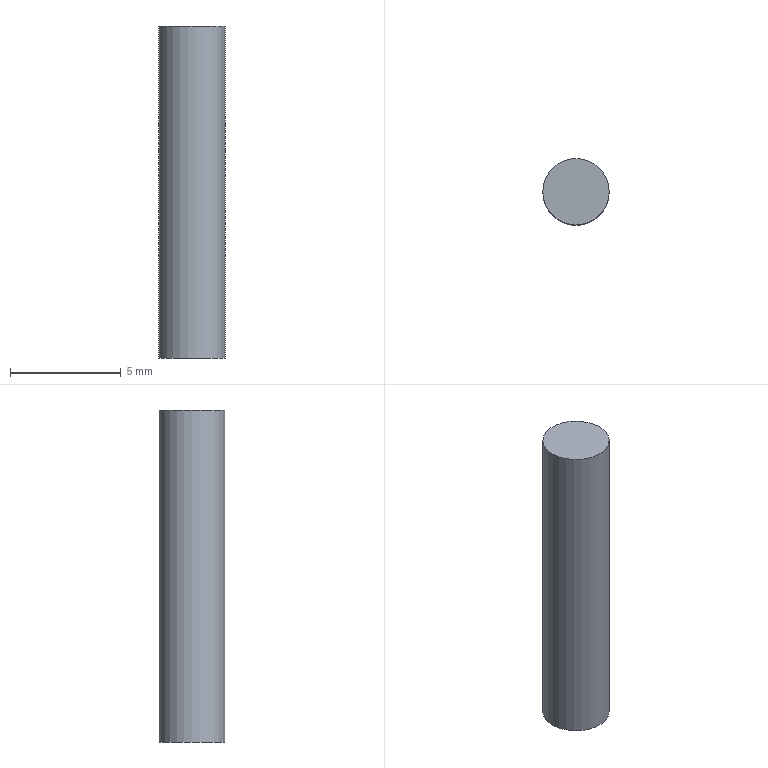Component | NX | 1_SMALL_SHAFT | 1 solid | 3 faces | box 3 x 3 x 15 mm | volume 106 mm3 | plane 2 | cylinder 1 | commonest cylinder face diameters 3 x1
STEP:
#1=CARTESIAN_POINT('',(0.,0.,0.));
#2=DIRECTION('',(0.,0.,1.));
#3=DIRECTION('',(1.,0.,0.));
#4=AXIS2_PLACEMENT_3D('',#1,#2,#3);
#5=CARTESIAN_POINT('',(-66.584,-165.706,-230.719));
#6=VERTEX_POINT('',#5);
#7=CARTESIAN_POINT('',(-68.084,-165.706,-230.719));
#8=DIRECTION('',(0.,0.,-1.));
#9=DIRECTION('',(1.,0.,0.));
#10=AXIS2_PLACEMENT_3D('',#7,#8,#9);
#11=CIRCLE('',#10,1.5);
#12=CARTESIAN_POINT('',(-68.084,-165.706,-230.719));
#13=DIRECTION('',(0.,0.,1.));
#14=DIRECTION('',(1.,0.,0.));
#15=AXIS2_PLACEMENT_3D('',#12,#13,#14);
#16=PLANE('',#15);
#17=CARTESIAN_POINT('',(1.5,0.));
#18=CARTESIAN_POINT('',(1.5,-2.598));
#19=CARTESIAN_POINT('',(-0.75,-1.299));
#20=CARTESIAN_POINT('',(-3.,-0.));
#21=CARTESIAN_POINT('',(-0.75,1.299));
#22=CARTESIAN_POINT('',(1.5,2.598));
#23=CARTESIAN_POINT('',(1.5,0.));
#24=(BOUNDED_CURVE()B_SPLINE_CURVE(2,(#17,#18,#19,#20,#21,#22,#23),.UNSPECIFIED.,.T.,.F.)B_SPLINE_CURVE_WITH_KNOTS((1,2,2,2,2,1),(-2.094,0.,2.094,4.189,6.283,8.378),.UNSPECIFIED.)CURVE()GEOMETRIC_REPRESENTATION_ITEM()RATIONAL_B_SPLINE_CURVE((1.,0.5,1.,0.5,1.,0.5,1.))REPRESENTATION_ITEM(''));
#25=(GEOMETRIC_REPRESENTATION_CONTEXT(2)PARAMETRIC_REPRESENTATION_CONTEXT()REPRESENTATION_CONTEXT('',''));
#26=DEFINITIONAL_REPRESENTATION('',(#24),#25);
#27=PCURVE('',#16,#26);
#28=CARTESIAN_POINT('',(-68.084,-165.706,-245.719));
#29=DIRECTION('',(0.,0.,1.));
#30=DIRECTION('',(1.,0.,0.));
#31=AXIS2_PLACEMENT_3D('',#28,#29,#30);
#32=CYLINDRICAL_SURFACE('',#31,1.5);
#33=CARTESIAN_POINT('',(6.283,15.));
#34=DIRECTION('',(-1.,0.));
#35=VECTOR('',#34,1.);
#36=LINE('',#33,#35);
#37=(GEOMETRIC_REPRESENTATION_CONTEXT(2)PARAMETRIC_REPRESENTATION_CONTEXT()REPRESENTATION_CONTEXT('',''));
#38=DEFINITIONAL_REPRESENTATION('',(#36),#37);
#39=PCURVE('',#32,#38);
#40=SURFACE_CURVE('',#11,(#27,#39),.PCURVE_S1.);
#41=EDGE_CURVE('',#6,#6,#40,.T.);
#42=ORIENTED_EDGE('',*,*,#41,.F.);
#43=EDGE_LOOP('',(#42));
#44=FACE_BOUND('',#43,.T.);
#45=ADVANCED_FACE('',(#44),#16,.T.);
#46=CARTESIAN_POINT('',(-66.584,-165.706,-245.719));
#47=VERTEX_POINT('',#46);
#48=CARTESIAN_POINT('',(-68.084,-165.706,-245.719));
#49=DIRECTION('',(0.,0.,1.));
#50=DIRECTION('',(1.,0.,0.));
#51=AXIS2_PLACEMENT_3D('',#48,#49,#50);
#52=CIRCLE('',#51,1.5);
#53=CARTESIAN_POINT('',(-68.084,-165.706,-245.719));
#54=DIRECTION('',(0.,0.,-1.));
#55=DIRECTION('',(-1.,0.,0.));
#56=AXIS2_PLACEMENT_3D('',#53,#54,#55);
#57=PLANE('',#56);
#58=CARTESIAN_POINT('',(-1.5,0.));
#59=CARTESIAN_POINT('',(-1.5,2.598));
#60=CARTESIAN_POINT('',(0.75,1.299));
#61=CARTESIAN_POINT('',(3.,0.));
#62=CARTESIAN_POINT('',(0.75,-1.299));
#63=CARTESIAN_POINT('',(-1.5,-2.598));
#64=CARTESIAN_POINT('',(-1.5,0.));
#65=(BOUNDED_CURVE()B_SPLINE_CURVE(2,(#58,#59,#60,#61,#62,#63,#64),.UNSPECIFIED.,.T.,.F.)B_SPLINE_CURVE_WITH_KNOTS((1,2,2,2,2,1),(-2.094,0.,2.094,4.189,6.283,8.378),.UNSPECIFIED.)CURVE()GEOMETRIC_REPRESENTATION_ITEM()RATIONAL_B_SPLINE_CURVE((1.,0.5,1.,0.5,1.,0.5,1.))REPRESENTATION_ITEM(''));
#66=(GEOMETRIC_REPRESENTATION_CONTEXT(2)PARAMETRIC_REPRESENTATION_CONTEXT()REPRESENTATION_CONTEXT('',''));
#67=DEFINITIONAL_REPRESENTATION('',(#65),#66);
#68=PCURVE('',#57,#67);
#69=CARTESIAN_POINT('',(0.,0.));
#70=DIRECTION('',(1.,0.));
#71=VECTOR('',#70,1.);
#72=LINE('',#69,#71);
#73=(GEOMETRIC_REPRESENTATION_CONTEXT(2)PARAMETRIC_REPRESENTATION_CONTEXT()REPRESENTATION_CONTEXT('',''));
#74=DEFINITIONAL_REPRESENTATION('',(#72),#73);
#75=PCURVE('',#32,#74);
#76=SURFACE_CURVE('',#52,(#68,#75),.PCURVE_S1.);
#77=EDGE_CURVE('',#47,#47,#76,.T.);
#78=ORIENTED_EDGE('',*,*,#77,.F.);
#79=EDGE_LOOP('',(#78));
#80=FACE_BOUND('',#79,.T.);
#81=ADVANCED_FACE('',(#80),#57,.T.);
#82=ORIENTED_EDGE('',*,*,#41,.T.);
#83=CARTESIAN_POINT('',(-66.584,-165.706,-245.719));
#84=CARTESIAN_POINT('',(-66.584,-165.706,-230.719));
#85=B_SPLINE_CURVE_WITH_KNOTS('',1,(#83,#84),.UNSPECIFIED.,.F.,.F.,(2,2),(0.,15.),.PIECEWISE_BEZIER_KNOTS.);
#86=CARTESIAN_POINT('',(0.,0.));
#87=DIRECTION('',(0.,1.));
#88=VECTOR('',#87,1.);
#89=LINE('',#86,#88);
#90=(GEOMETRIC_REPRESENTATION_CONTEXT(2)PARAMETRIC_REPRESENTATION_CONTEXT()REPRESENTATION_CONTEXT('',''));
#91=DEFINITIONAL_REPRESENTATION('',(#89),#90);
#92=PCURVE('',#32,#91);
#93=CARTESIAN_POINT('',(6.283,0.));
#94=DIRECTION('',(0.,1.));
#95=VECTOR('',#94,1.);
#96=LINE('',#93,#95);
#97=(GEOMETRIC_REPRESENTATION_CONTEXT(2)PARAMETRIC_REPRESENTATION_CONTEXT()REPRESENTATION_CONTEXT('',''));
#98=DEFINITIONAL_REPRESENTATION('',(#96),#97);
#99=PCURVE('',#32,#98);
#100=SEAM_CURVE('',#85,(#92,#99),.PCURVE_S1.);
#101=EDGE_CURVE('',#47,#6,#100,.T.);
#102=ORIENTED_EDGE('',*,*,#101,.F.);
#103=ORIENTED_EDGE('',*,*,#77,.T.);
#104=ORIENTED_EDGE('',*,*,#101,.T.);
#105=EDGE_LOOP('',(#82,#102,#103,#104));
#106=FACE_BOUND('',#105,.T.);
#107=ADVANCED_FACE('',(#106),#32,.T.);
#108=CLOSED_SHELL('',(#45,#81,#107));
#109=MANIFOLD_SOLID_BREP('',#108);
#110=(LENGTH_UNIT()NAMED_UNIT(*)SI_UNIT(.MILLI.,.METRE.));
#111=UNCERTAINTY_MEASURE_WITH_UNIT(LENGTH_MEASURE(0.00001),#110,'','');
#112=(NAMED_UNIT(*)PLANE_ANGLE_UNIT()SI_UNIT($,.RADIAN.));
#113=(NAMED_UNIT(*)SI_UNIT($,.STERADIAN.)SOLID_ANGLE_UNIT());
#114=(GEOMETRIC_REPRESENTATION_CONTEXT(3)GLOBAL_UNCERTAINTY_ASSIGNED_CONTEXT((#111))GLOBAL_UNIT_ASSIGNED_CONTEXT((#110,#112,#113))REPRESENTATION_CONTEXT('',''));
#115=ADVANCED_BREP_SHAPE_REPRESENTATION('',(#4,#109),#114);